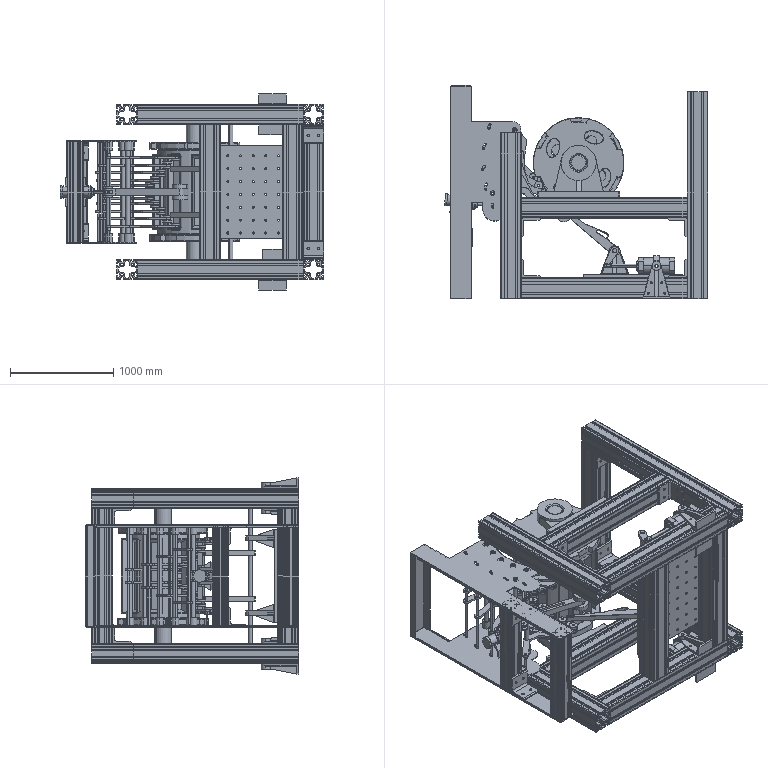Assembly | SolidWorks | mm | 107 component files | 109 solids | 5082 faces | box 2545.98 x 2062 x 1896 mm | volume 839477770 mm3 | plane 3158 | cylinder 1371 | cone 332 | spline 113 | torus 100 | sphere 8 | commonest cylinder face diameters 20 x420 12 x132 24 x88 44.189 x76 60 x61 4 x48 10 x44 85 x40
Bill of materials:
AluminumIngotContainer | 10 |  | Elongated straight prism with a four-sided, non-rectangular (trapezoid/parallelogram-like) cross-section; plain flat faces with no holes or cutouts.
AluminumProfile | 2 |  | Straight extruded bar with a square, slotted profile: two undercut T-style slots on each side, four round bores in the inner lobes, small round corner channels with narrow slits, and a large cross-shaped central cavity.
AluminumProfile100x100 | 6 |  | Straight extruded bar with the same square, slotted profile: two undercut slots per side, four round inner bores, four small corner channels and a cross-shaped central cavity.
AluminumProfile2 | 3 |  | Straight square extruded bar with two undercut slots on each side, four round inner bores, small corner channels and a cross-shaped central cavity; shown standing vertically.
AluminumProfile3 | 2 |  | Straight square extruded bar with two undercut slots on each side, four round inner bores, small corner channels and a cross-shaped central cavity; shown standing vertically.
ConnectingRod1 | 2 | 45 | Flat, thick tapered link plate with rounded ends: a large through-hole in the wide end and a small through-hole in the narrow end.
Cylinder2 | 1 |  | Stepped cylindrical part (shaft or sleeve) with an axial bore. It has end collars, a raised central collar with a radial cross-hole, and a stepped spigot at one end. The bore looks D-shaped, with a flat.
CylinderPistonRod | 2 | 45 | Slender round rod with a flattened eye end (small through-hole) at one end and a larger solid cylindrical head at the other.
cz | 2 |  | Thick circular disc with a small central through-hole and small chamfers on the outer edges and the hole edge.
IngotConnectingArm | 2 | 45 | Flat, elongated, tapered lever plate. It has a rounded boss end with a pivot through-hole, a small radial hole into the boss edge, a triangular through-slot, and a small rectangular tab standing up from one edge.
IngotConnectingRodMandrel | 4 |  | Very long, slender cylindrical rod or tube. The end view shows a central faceted feature that may be a small axial bore or a conical end recess.
IngotSupportRod | 10 | 45 | Thin flat bent link (bell-crank-like) plate with three arm segments, rounded ends, a small hole at each end, and a larger hole at the corner between the first two arms.
Mandrel | 6 | 45 | Long slender cylindrical rod with an enlarged cylindrical collar at each end and a short smaller stub beyond each collar; the end view shows an annular face with a central axial hole.
Mandrel2 | 1 | 45 | Plain solid slender cylindrical rod of uniform diameter with flat ends.
MiddleTrunnionCylinder | 2 | 45 | Axisymmetric body with octagonal prism sections at both ends and a larger octagonal collar in the middle, joined by cylindrical sections, plus a short chamfered cylindrical spigot at one end. A single radial cross-hole passes through the central collar.
MountingPlate | 1 | 45 | Thin flat rectangular plate with a regular grid of small round through holes: 7 rows, where the five inner rows have 9 holes and the top and bottom rows have 7 holes (the two right-hand columns are missing in those rows).
Piston2 | 1 |  | Stepped pin with a larger cylindrical head, a long slender cylindrical shank, and a rounded tip end with a transverse through hole.
Roller | 20 | 45 | Thick circular disc or washer-like ring with a central through hole and chamfered outer edges on both faces.
SmallPin | 2 |  | Stepped cylindrical shaft with a long shank, a larger-diameter collar near one end, and a short smaller stub beyond the collar. The stub end face has a small central hole.
SupportBase | 2 | 45 | Bracket made of a rectangular mounting flange with four small through holes near its ends, and a perpendicular tapered lug with a rounded end and one large through hole.
SupportBase2 | 2 |  | Bracket with a flat rectangular back plate and a perpendicular tapered, pocketed lug. The lug has a raised perimeter rim, a central rib, and a rounded boss at the apex with a through hole.
SupportBase3 | 2 |  | Tapered triangular plate bracket with a rounded apex holding a larger through hole, four smaller through holes in two pairs, and a perpendicular flange along the wide base edge.
SupportBase3 | 1 |  | L-shaped bracket. A flat, symmetric, tapered (trapezoidal) base plate has a wide end and a narrow end with a rounded tip. A rectangular vertical flange rises along the full width of the wide end. A raised central rib runs along the plate's centerline and slopes down from the flange to a thicker cylindrical boss at the narrow end. The boss has a through hole. There are four smaller through holes in the plate, two on each side of the rib.
SupportBase3 | 1 |  | Asymmetric tapered plate bracket. It is a flat plate with one straight side and one angled side, narrowing to a rounded tip. The tip carries a larger through hole in a cylindrical boss that is deeper than the plate. A narrow flange turns down along the wide end. There are four smaller through holes in the plate. The side view suggests a tapered web or gusset under the plate, running from the flange to the boss.
SupportBase4 | 2 |  | Triangular gusset-style bracket: a triangular plate with a rounded apex and one through hole, joined at its base to a perpendicular rectangular flange that has two through holes.
SupportFrame | 1 |  | Thin-walled C-shaped frame: two parallel long thin strips joined at one end by a perpendicular web. Each strip has a lobed side extension with a concave curved edge, a row of round holes, and a row of short arc-shaped slots.
TappingArm | 1 |  | Long, flat, straight lever arm. One end has a cylindrical hub with a through bore, and a forked side lug extends from that end at an angle. The arm has a long slot along its length and a small hole near its rounded far end.
U-shapedPlate | 12 |  | L-section angle bracket with two legs of similar length at 90 degrees. It has a rounded inner bend, slightly rounded outer corner and chamfered leg tips. Each leg has two round through-holes in a line.
Wheel | 1 | 45 | Short solid cylinder with a central axial bore and four smaller axial through-holes evenly spaced on a bolt circle. The outer surface has longitudinal rectangular recessed pockets around its circumference, and the end edges are chamfered.
WheelIndexingPlate | 2 | 45 | Thin flat disc with a stepped, notched outer edge, a central round hole, and four oval through-holes arranged around the center.
WheelMandrel | 1 |  | Plain solid straight cylindrical rod or pin with small chamfers at both ends.
Mates:
1. coincident | SupportFrame-2 plane at (0, 0, 0) dir (0, 0, 1) | assembly plane at (0, 0, 0) dir (0, 0, 1)
2. coincident | SupportFrame-2 plane at (0, 0, 0) dir (0, 1, 0) | assembly plane at (0, 0, 0) dir (0, 1, 0)
3. coincident | SupportFrame-2 plane at (0, 0, 0) dir (1, 0, 0) | assembly plane at (0, 0, 0) dir (1, 0, 0)
4. width | Wheel-1 face at (1138.564, 280.356, 80) dir (0, 0, -1) | Wheel-1 face at (1138.564, 280.356, 910) dir (0, 0, 1) | SupportFrame-2 face at (0, 0, 0) dir (0, 0, -1) | SupportFrame-2 face at (0, 0, 990) dir (0, 0, 1)
5. concentric | SupportFrame-2 face at (521.144, 598.058, -1429) dir (0, 0, 1) r 22.094 | Mandrel-1 face at (521.144, 598.058, 995) dir (0, 0, -1) r 22.094
6. width | Mandrel-1 face at (521.144, 598.058, -5) dir (0, 0, -1) | Mandrel-1 face at (521.144, 598.058, 995) dir (0, 0, 1) | SupportFrame-2 face at (0, 0, 990) dir (0, 0, 1) | SupportFrame-2 face at (0, 0, 0) dir (0, 0, -1)
7. concentric | Wheel-1 face at (1138.564, 280.356, -180) dir (0, 0, 1) r 80 | SupportBase-1 face at (1138.564, 280.356, -155) dir (0, 0, -1) r 80
8. concentric | Mandrel-1 face at (521.144, 598.058, 995) dir (0, 0, -1) r 22.094 | IngotSupportRod-1 face at (521.144, 598.058, 445) dir (0, 0, -1) r 22.094
9. concentric | IngotSupportRod-1 face at (705.127, 143.342, 445) dir (0, 0, -1) r 30 | Roller-2 face at (705.127, 143.342, 470) dir (0, 0, -1) r 10
10. concentric | IngotSupportRod-1 face at (705.127, 143.342, 445) dir (0, 0, -1) r 30 | Roller-1 face at (705.127, 143.342, 425) dir (0, 0, -1) r 10
11. coincident | IngotSupportRod-1 face at (17.945, 67.185, 425) dir (0, 0, -1) | Roller-1 face at (705.127, 143.342, 425) dir (0, 0, 1)
12. coincident | IngotSupportRod-1 face at (17.945, 67.185, 445) dir (0, 0, 1) | Roller-2 face at (705.127, 143.342, 445) dir (0, 0, -1)
13. concentric | Mandrel-4 face at (440.739, 312.216, 995) dir (0, 0, -1) r 22.094 | IngotSupportRod-5 face at (440.739, 312.216, 320) dir (0, 0, -1) r 22.094
14. concentric | Mandrel-5 face at (450.613, 163.114, 995) dir (0, 0, -1) r 22.094 | IngotSupportRod-6 face at (450.613, 163.114, 245) dir (0, 0, -1) r 22.094
15. concentric | Mandrel-6 face at (493.776, 20.056, 995) dir (0, 0, -1) r 22.094 | IngotSupportRod-7 face at (493.776, 20.056, 170) dir (0, 0, -1) r 22.094
16. concentric | Roller-3 face at (753.229, 63.053, 370) dir (0, 0, -1) r 10 | IngotSupportRod-4 face at (753.229, 63.053, 390) dir (0, 0, -1) r 10
17. coincident | Roller-3 face at (753.229, 63.053, 370) dir (0, 0, 1) | IngotSupportRod-4 face at (104.912, -177.165, 370) dir (0, 0, -1)
18. concentric | Roller-3 face at (753.229, 63.053, 370) dir (0, 0, -1) r 42.5 | Roller-7 face at (753.229, 63.053, 415) dir (0, 0, -1) r 42.5
19. coincident | Roller-7 face at (753.229, 63.053, 390) dir (0, 0, -1) | IngotSupportRod-4 face at (104.912, -177.165, 390) dir (0, 0, 1)
20. concentric | Roller-4 face at (809.993, -10.688, 345) dir (0, 0, -1) r 42.5 | Roller-8 face at (809.993, -10.688, 300) dir (0, 0, -1) r 42.5
21. concentric | Roller-4 face at (809.993, -10.688, 345) dir (0, 0, -1) r 42.5 | IngotSupportRod-5 face at (809.993, -10.688, 320) dir (0, 0, -1) r 30
22. coincident | Roller-4 face at (809.993, -10.688, 320) dir (0, 0, -1) | IngotSupportRod-5 face at (230.978, -388.524, 320) dir (0, 0, 1)
23. coincident | Roller-8 face at (809.993, -10.688, 300) dir (0, 0, 1) | IngotSupportRod-5 face at (230.978, -388.524, 300) dir (0, 0, -1)
24. concentric | Roller-5 face at (870.434, -90.592, 270) dir (0, 0, -1) r 10 | IngotSupportRod-6 face at (870.434, -90.592, 245) dir (0, 0, -1) r 30
25. coincident | Roller-5 face at (870.434, -90.592, 245) dir (0, 0, -1) | IngotSupportRod-6 face at (366.019, -563.439, 245) dir (0, 0, 1)
26. concentric | Roller-9 face at (870.434, -90.592, 225) dir (0, 0, -1) r 10 | IngotSupportRod-6 face at (870.434, -90.592, 245) dir (0, 0, -1) r 30
27. coincident | Roller-9 face at (870.434, -90.592, 225) dir (0, 0, 1) | IngotSupportRod-6 face at (366.019, -563.439, 225) dir (0, 0, -1)
28. concentric | Roller-6 face at (950.087, -159.933, 195) dir (0, 0, -1) r 42.5 | Roller-10 face at (950.087, -159.933, 150) dir (0, 0, -1) r 42.5
29. concentric | Roller-6 face at (950.087, -159.933, 195) dir (0, 0, -1) r 42.5 | IngotSupportRod-7 face at (950.087, -159.933, 170) dir (0, 0, -1) r 30
30. coincident | Roller-6 face at (950.087, -159.933, 170) dir (0, 0, -1) | IngotSupportRod-7 face at (531.776, -710.418, 170) dir (0, 0, 1)
31. coincident | Roller-10 face at (950.087, -159.933, 150) dir (0, 0, 1) | IngotSupportRod-7 face at (531.776, -710.418, 150) dir (0, 0, -1)
32. concentric | Wheel-1 face at (1138.564, 280.356, -180) dir (0, 0, 1) r 80 | WheelIndexingPlate-1 face at (1138.564, 280.356, 80) dir (0, 0, -1) r 80
33. coincident | Wheel-1 face at (1138.564, 280.356, 80) dir (0, 0, -1) | WheelIndexingPlate-1 face at (1138.564, 280.356, 80) dir (0, 0, 1)
34. concentric | Mandrel-3 face at (464.658, 459.717, 995) dir (0, 0, -1) r 22.094 | IngotSupportRod-4 face at (464.658, 459.717, 390) dir (0, 0, -1) r 22.094
35. concentric | Wheel-1 face at (1138.564, 280.356, 910) dir (0, 0, -1) r 357.5 | WheelIndexingPlate-3 face at (1138.564, 280.356, 970) dir (0, 0, -1) r 395
36. coincident | Wheel-1 face at (1138.564, 280.356, 910) dir (0, 0, 1) | WheelIndexingPlate-3 face at (1138.564, 280.356, 910) dir (0, 0, -1)
37. coincident | Wheel-1 face at (925.229, 626.929, 135) dir (-0.9256, -0.3784, 0) | AluminumIngotContainer-1 face at (925.229, 626.929, 135) dir (0.9256, 0.3784, 0)
38. coincident | Wheel-1 face at (919.439, 521.727, 80) dir (-0.6722, 0.7404, 0) | AluminumIngotContainer-1 face at (919.439, 521.727, 495) dir (0.6722, -0.7404, 0)
39. coincident | Wheel-1 face at (925.229, 626.929, 855) dir (-0.2299, 0.2532, -0.9397) | AluminumIngotContainer-1 face at (814.168, 526.105, 855) dir (0.2299, -0.2532, 0.9397)
40. concentric | MiddleTrunnionCylinder-1 face at (1766, -713.926, -260) dir (-1, 0.0005394, 0) r 40 | CylinderPistonRod-1 face at (1749.707, -713.917, -260) dir (1, -0.0005394, 0) r 40
41. parallel | MiddleTrunnionCylinder-1 face at (1765.96, -788.926, -335) dir (0, 0, -1) | CylinderPistonRod-1 face at (1399.707, -713.728, -280) dir (0, 0, -1)
42. concentric | CylinderPistonRod-1 face at (1399.707, -713.728, -280) dir (0, 0, 1) r 8.5 | ConnectingRod1-1 face at (1399.707, -713.728, -200) dir (0, 0, -1) r 8.5
43. distance | IngotSupportRod-1 face at (17.945, 67.185, 445) dir (0, 0, 1) | IngotSupportRod-13 face at (17.945, 67.185, 545) dir (0, 0, -1)
44. distance | IngotSupportRod-4 face at (104.912, -177.165, 390) dir (0, 0, 1) | IngotSupportRod-12 face at (104.912, -177.165, 600) dir (0, 0, -1)
45. distance | IngotSupportRod-5 face at (230.978, -388.524, 320) dir (0, 0, 1) | IngotSupportRod-16 face at (230.978, -388.524, 670) dir (0, 0, -1)
46. distance | IngotSupportRod-6 face at (366.019, -563.439, 245) dir (0, 0, 1) | IngotSupportRod-15 edge at (458.04, 192.181, 745) dir (0.9689, -0.2475, 0)
47. distance | IngotSupportRod-7 face at (531.776, -710.418, 170) dir (0, 0, 1) | IngotSupportRod-14 face at (531.776, -710.418, 820) dir (0, 0, -1)
48. coincident | CylinderPistonRod-1 face at (1399.707, -713.728, -240) dir (0, 0, 1) | ConnectingRod1-1 face at (468.852, 496.589, -240) dir (0, 0, -1)
49. concentric | ConnectingRod1-1 face at (1486.2, -567.376, -200) dir (0, 0, -1) r 21.5 | Mandrel2-1 face at (1486.2, -567.376, 748.53) dir (0, 0, -1) r 21.5
50. concentric | Mandrel2-1 face at (1486.2, -567.376, 748.53) dir (0, 0, -1) r 21.5 | IngotConnectingArm-1 face at (1486.2, -567.376, 297.813) dir (0, 0, -1) r 21.5
51. coincident | AluminumProfile100x100-1 face at (2186, -968.8, -155) dir (0, 0, 1) | AluminumProfile100x100-3 face at (2186, -190.8, -155) dir (0, 0, 1)
52. coincident | AluminumProfile100x100-2 face at (448.2, 569, -355) dir (0, 0, -1) | AluminumProfile100x100-3 face at (2186, -115.2, -355) dir (0, 0, -1)
53. coincident | AluminumProfile100x100-2 face at (586, 569, -292.8) dir (1, 0, 0) | AluminumProfile100x100-3 face at (586, -248, -350) dir (-1, 0, 0)
54. coincident | AluminumProfile100x100-1 face at (586, -1026, -160) dir (-1, 0, 0) | AluminumProfile100x100-2 face at (586, 569, -292.8) dir (1, 0, 0)
55. coincident | SupportFrame-2 face at (100, -1031, 10) dir (0, -1, 0) | AluminumProfile100x100-2 face at (391, -1031, -350) dir (0, -1, 0)
56. parallel | SupportFrame-2 face at (100, -1031, 10) dir (0, -1, 0) | SupportBase-1 face at (138.564, -53, -155) dir (0, -1, 0)
57. coincident | SupportBase-1 face at (138.564, -53, -155) dir (0, -1, 0) | AluminumProfile100x100-3 face at (2186, -53, -217.2) dir (0, 1, 0)
58. coincident | SupportBase-1 face at (138.564, 0.2627, -155) dir (0, 0, 1) | AluminumProfile100x100-3 face at (2186, -90.8, -155) dir (0, 0, 1)
59. distance | Wheel-1 plane at (1138.564, 280.356, 495) dir (0, 0, 1) | AluminumProfile100x100-3 face at (2186, -190.8, -155) dir (0, 0, 1)
60. coincident | AluminumProfile100x100-1 face at (2186, -1026, -160) dir (1, 0, 0) | AluminumProfile-1 face at (2186, 969, -217.2) dir (-1, 0, 0)
61. coincident | AluminumProfile100x100-1 face at (2186, -1031, -292.8) dir (0, -1, 0) | AluminumProfile-1 face at (2191, -1031, -350) dir (0, -1, 0)
62. coincident | AluminumProfile100x100-1 face at (2186, -1031, -292.8) dir (0, -1, 0) | AluminumProfile2-1 face at (2123.8, -1031, 1145) dir (0, -1, 0)
63. coincident | AluminumProfile100x100-5 face at (2186, -1031, 1207.2) dir (0, -1, 0) | AluminumProfile100x100-6 face at (391, -1031, 1150) dir (0, -1, 0)
64. coincident | AluminumProfile100x100-5 face at (2186, -893.2, 1145) dir (0, 0, -1) | AluminumProfile2-1 face at (1991, -1026, 1145) dir (0, 0, 1)
65. coincident | MiddleTrunnionCylinder-1 face at (1915.976, -759.007, -355) dir (0, 0, -1) | AluminumProfile100x100-1 face at (2186, -893.2, -355) dir (0, 0, -1)
66. coincident | MountingPlate-1 face at (-545.911, -831, -80.281) dir (0, -1, 0) | AluminumProfile2-1 face at (2048.2, -831, 1145) dir (0, 1, 0)
67. coincident | MountingPlate-1 face at (2186, -801, 45) dir (1, 0, 0) | AluminumProfile2-1 face at (2186, -893.2, 1145) dir (1, 0, 0)
68. distance | SupportBase-1 face at (742.414, 0.2627, -155) dir (-1, 0, 0) | AluminumProfile100x100-2 face at (586, 569, -292.8) dir (1, 0, 0)
69. coincident | AluminumProfile100x100-3 face at (2186, -115.2, -355) dir (0, 0, -1) | AluminumProfile-1 face at (2248.2, 969, -355) dir (0, 0, -1)
70. distance | SupportBase-1 face at (138.564, -53, -155) dir (0, -1, 0) | AluminumProfile100x100-1 face at (2186, -1031, -292.8) dir (0, -1, 0)
71. coincident | AluminumProfile100x100-1 face at (2186, -968.8, -155) dir (0, 0, 1) | AluminumProfile2-2 face at (1191, -836, -155) dir (0, 0, -1)
72. coincident | AluminumProfile100x100-1 face at (2186, -1031, -292.8) dir (0, -1, 0) | AluminumProfile2-2 face at (1323.8, -1031, 1145) dir (0, -1, 0)
73. coincident | MountingPlate-1 face at (1186, -801, 45) dir (-1, 0, 0) | AluminumProfile2-2 face at (1186, -968.8, 1145) dir (-1, 0, 0)
74. coincident | AluminumProfile-1 face at (2186, 969, -217.2) dir (-1, 0, 0) | AluminumProfile2-1 face at (2186, -893.2, 1145) dir (1, 0, 0)
75. coincident | MountingPlate-1 face at (-545.911, -801, -80.281) dir (0, 1, 0) | SupportBase2-2 face at (165.227, -801, 120) dir (0, -1, 0)
76. concentric | Mandrel2-1 face at (1486.2, -567.376, 748.53) dir (0, 0, -1) r 21.5 | SupportBase2-2 face at (1486.2, -567.376, 120) dir (0, 0, 1) r 21.5
77. coincident | MountingPlate-1 face at (2186, -801, 45) dir (0, 0, -1) | SupportBase2-2 face at (165.227, 0, 45) dir (0, 0, -1)
78. distance | AluminumProfile100x100-2 face at (386, 569, -217.2) dir (-1, 0, 0) | SupportFrame-2 face at (-100, 1031, 10) dir (-1, 0, 0)
79. width | AluminumProfile100x100-1 face at (2186, -893.2, -355) dir (0, 0, -1) | AluminumProfile100x100-5 face at (2186, -968.8, 1345) dir (0, 0, 1) | MountingPlate-1 face at (2186, -801, 45) dir (0, 0, -1) | MountingPlate-1 face at (2186, -801, 945) dir (0, 0, 1)
80. distance | AluminumProfile2-2 face at (1346.2, -841, 1145) dir (-1, 0, 0) | SupportBase2-2 face at (1466.2, -659.188, 133) dir (-1, 0, 0)
81. coincident | AluminumProfile100x100-1 face at (2186, -1031, -292.8) dir (0, -1, 0) | SupportBase3-1 face at (1336.2, -1031, -375) dir (0, -1, 0)
82. concentric | MiddleTrunnionCylinder-1 face at (1891, -713.993, -415) dir (0, 0, 1) r 15 | SupportBase3-1 face at (1891, -713.993, -375) dir (0, 0, 1) r 15
83. distance | SupportBase3-1 face at (1906, -850.78, -404) dir (1, 0, 0) | AluminumProfile-1 face at (2386, 969, -292.8) dir (1, 0, 0)
84. parallel | ConnectingRod1-1 face at (1675.336, -366.804, -200) dir (0.8132, -0.582, 0) | IngotConnectingArm-1 face at (1107.928, -241.338, 297.813) dir (0.8132, -0.582, 0)
85. concentric | MiddleTrunnionCylinder-1 face at (1891, -713.993, -415) dir (0, 0, 1) r 15 | SupportBase3-2 face at (1891, -713.993, -135) dir (0, 0, -1) r 15
86. coincident | AluminumProfile100x100-1 face at (2186, -1031, -292.8) dir (0, -1, 0) | SupportBase3-2 face at (2445.8, -1031, -135) dir (0, -1, 0)
87. coincident | AluminumProfile100x100-1 face at (2186, -1026, -155) dir (0, 0, 1) | SupportBase3-2 face at (2445.8, -908.993, -155) dir (0, 0, -1)
88. concentric | Mandrel2-1 face at (1492.399, -572.235, 272.813) dir (-0.7871, 0.6169, 0) r 8 | IngotConnectingArm-1 face at (1521.618, -595.136, 272.813) dir (0.7871, -0.6169, 0) r 8
89. width | AluminumProfile100x100-5 face at (2186, -968.8, 1345) dir (0, 0, 1) | AluminumProfile100x100-1 face at (2186, -893.2, -355) dir (0, 0, -1) | Mandrel2-1 face at (1486.2, -567.376, -248.47) dir (0, 0, -1) | Mandrel2-1 face at (1486.2, -567.376, 1238.47) dir (0, 0, 1)
90. distance | CylinderPistonRod-1 face at (1799.707, -713.944, -260) dir (1, -0.0005394, 0) | MiddleTrunnionCylinder-1 face at (2016.387, 2.939, -1754.26) dir (-1, 0.0005394, 0)
91. coincident | AluminumProfile100x100-1 face at (2186, -893.2, -355) dir (0, 0, -1) | SupportBase3-1 face at (1336.2, -908.993, -355) dir (0, 0, 1)
92. coincident | SupportFrame-2 face at (0, 0, 980) dir (0, 0, -1) | AluminumProfile3-1 face at (-86.25, -203.572, 980) dir (0, 0, 1)
93. coincident | SupportFrame-2 face at (-90, 926.986, 20) dir (1, 0, 0) | AluminumProfile3-1 face at (-90, -303.172, 980) dir (-1, 0, 0)
94. distance | SupportFrame-2 face at (90, -119.822, 20) dir (0, 1, 0) | AluminumProfile3-1 face at (31.65, -199.822, 980) dir (0, 1, 0)
95. coincident | SupportFrame-2 face at (0, 0, 10) dir (0, 0, 1) | AluminumProfile3-2 face at (-86.25, -884.75, 10) dir (0, 0, -1)
96. coincident | SupportFrame-2 face at (-90, 926.986, 20) dir (1, 0, 0) | AluminumProfile3-2 face at (-90, -984.35, 980) dir (-1, 0, 0)
97. coincident | SupportFrame-2 face at (100, -1031, 10) dir (0, -1, 0) | AluminumProfile3-2 face at (13.35, -1031, 980) dir (0, -1, 0)
98. coincident | AluminumProfile3-1 face at (-43.35, -199.822, 980) dir (0, 1, 0) | SupportBase4-1 face at (19.647, -199.822, 632.958) dir (0, -1, 0)
99. concentric | Cylinder2-1 face at (-15, -91.375, 405) dir (0, 0, 1) r 11.5 | SupportBase4-1 face at (-15, -91.375, 437.28) dir (0, 0, -1) r 11.5
100. width | AluminumProfile3-1 face at (-90, -303.172, 980) dir (-1, 0, 0) | AluminumProfile3-1 face at (60, -246.472, 980) dir (1, 0, 0) | SupportBase4-1 face at (-25, -130.511, 397.53) dir (-1, 0, 0) | SupportBase4-1 face at (-5, -130.511, 397.53) dir (1, 0, 0)
101. concentric | Cylinder2-1 face at (144.994, -111.29, 495) dir (-0.9923, 0.1235, 0) r 50 | Piston2-1 face at (257.687, -125.317, 495) dir (-0.9923, 0.1235, 0) r 15
102. concentric | SupportFrame-2 face at (306.906, -12.931, 990) dir (0, 0, -1) r 22.095 | Mandrel-7 face at (306.906, -12.931, 995) dir (0, 0, -1) r 22.094
103. coincident | SupportFrame-2 face at (0, 0, 980) dir (0, 0, -1) | Mandrel-7 face at (306.906, -12.931, 980) dir (0, 0, 1)
104. concentric | TappingArm-1 face at (306.906, -12.931, 525) dir (0, 0, -1) r 22.095 | Mandrel-7 face at (306.906, -12.931, 995) dir (0, 0, -1) r 22.094
105. concentric | Piston2-1 face at (302.342, -130.875, 510) dir (0, 0, -1) r 8 | TappingArm-1 face at (302.342, -130.875, 525) dir (0, 0, -1) r 8
106. coincident | Piston2-1 face at (302.342, -130.875, 510) dir (0, 0, 1) | TappingArm-1 face at (4.467, 40.819, 510) dir (0, 0, -1)
107. width | SupportFrame-2 face at (0, 0, 990) dir (0, 0, 1) | SupportFrame-2 face at (0, 0, 0) dir (0, 0, -1) | SupportBase4-1 face at (19.647, -70.838, 412.28) dir (0, 0, -1) | SupportBase4-2 face at (-49.647, -70.838, 577.72) dir (0, 0, 1)
108. concentric | TappingArm-1 face at (997.956, -215.048, 525) dir (0, 0, -1) r 36 | cz-1 face at (997.956, -215.048, 465) dir (0, 0, -1) r 75
109. coincident | TappingArm-1 face at (4.467, 40.819, 465) dir (0, 0, -1) | cz-1 face at (997.956, -215.048, 465) dir (0, 0, 1)
110. concentric | TappingArm-1 face at (997.956, -215.048, 525) dir (0, 0, -1) r 36 | cz-2 face at (997.956, -215.048, 571) dir (0, 0, -1) r 75
111. coincident | TappingArm-1 face at (4.467, 40.819, 525) dir (0, 0, 1) | cz-2 face at (997.956, -215.048, 525) dir (0, 0, -1)
112. coincident | AluminumProfile-1 face at (2191, 969, -350) dir (0, 1, 0) | AluminumProfile2-4 face at (2248.2, 969, 1145) dir (0, 1, 0)
113. coincident | AluminumProfile-1 face at (2386, 969, -292.8) dir (1, 0, 0) | AluminumProfile2-4 face at (2386, 906.8, 1145) dir (1, 0, 0)
114. coincident | AluminumProfile-1 face at (2323.8, 969, -155) dir (0, 0, 1) | AluminumProfile2-4 face at (2191, 774, -155) dir (0, 0, -1)
115. concentric | SupportBase-2 face at (1138.564, 280.356, 1145) dir (0, 0, 1) r 80 | WheelMandrel-1 face at (1138.564, 280.356, -255) dir (0, 0, 1) r 80
116. width | SupportBase-1 face at (1138.564, 280.356, -265) dir (0, 0, -1) | SupportBase-2 face at (1138.564, 280.356, 1255) dir (0, 0, 1) | WheelMandrel-1 face at (1138.564, 280.356, -255) dir (0, 0, -1) | WheelMandrel-1 face at (1138.564, 280.356, 1245) dir (0, 0, 1)
117. slot | IngotConnectingRodMandrel-1 face at (271.039, 615.177, -1.5) dir (0, 0, 1) r 10 | SupportFrame-2 face at (335.837, 614.405, 1660) dir (0, 0, -1) r 53.682
118. concentric | IngotSupportRod-1 face at (271.039, 615.177, 425) dir (0, 0, 1) r 10 | IngotConnectingRodMandrel-1 face at (271.039, 615.177, -1.5) dir (0, 0, 1) r 10
119. width | IngotConnectingRodMandrel-1 face at (271.039, 615.177, -1.5) dir (0, 0, -1) | IngotConnectingRodMandrel-1 face at (271.039, 615.177, 991.5) dir (0, 0, 1) | SupportFrame-2 face at (0, 0, 990) dir (0, 0, 1) | SupportFrame-2 face at (0, 0, 0) dir (0, 0, -1)
120. concentric | SupportFrame-2 face at (217.846, 415.792, 1660) dir (0, 0, -1) r 10.524 | IngotConnectingRodMandrel-2 face at (217.846, 415.792, 0) dir (0, 0, 1) r 10
121. coincident | SupportFrame-2 face at (0, 0, 0) dir (0, 0, -1) | IngotConnectingRodMandrel-2 face at (217.846, 415.792, 0) dir (0, 0, -1)
122. concentric | SupportFrame-2 face at (209.784, 214.72, 1660) dir (0, 0, -1) r 10.015 | IngotConnectingRodMandrel-3 face at (209.784, 214.72, 0) dir (0, 0, 1) r 10
123. coincident | SupportFrame-2 face at (0, 0, 0) dir (0, 0, -1) | IngotConnectingRodMandrel-3 face at (209.784, 214.72, 0) dir (0, 0, -1)
124. coincident | SupportFrame-2 face at (0, 0, 0) dir (0, 0, -1) | IngotConnectingRodMandrel-4 face at (240.154, 26.908, 0) dir (0, 0, -1)
125. concentric | SupportFrame-2 face at (240.154, 26.908, 1660) dir (0, 0, -1) r 10.764 | IngotConnectingRodMandrel-4 face at (240.154, 26.908, 993) dir (0, 0, -1) r 10
126. coincident | AluminumProfile-1 face at (2186, 969, -217.2) dir (-1, 0, 0) | U-shapedPlate-1 face at (2186, -433, -155) dir (1, 0, 0)
127. coincident | AluminumProfile-1 face at (2191, 969, -355) dir (0, 0, -1) | U-shapedPlate-1 face at (2146, -293, -355) dir (0, 0, -1)
128. coincident | AluminumProfile100x100-3 face at (2186, -253, -292.8) dir (0, -1, 0) | U-shapedPlate-1 face at (2186, -253, -155) dir (0, 1, 0)
129. coincident | AluminumProfile2-4 face at (2386, 906.8, 1145) dir (1, 0, 0) | U-shapedPlate-3 face at (2386, 729, -115) dir (1, 0, 0)
130. coincident | AluminumProfile2-4 face at (2323.8, 769, 1145) dir (0, -1, 0) | U-shapedPlate-3 face at (2386, 769, -155) dir (0, 1, 0)
131. coincident | AluminumProfile-1 face at (2323.8, 969, -155) dir (0, 0, 1) | U-shapedPlate-3 face at (2386, 589, -155) dir (0, 0, -1)
132. coincident | AluminumProfile100x100-2 face at (586, 569, -292.8) dir (1, 0, 0) | U-shapedPlate-4 face at (586, -433, -355) dir (-1, 0, 0)
133. coincident | AluminumProfile100x100-3 face at (2186, -253, -292.8) dir (0, -1, 0) | U-shapedPlate-4 face at (586, -253, -355) dir (0, 1, 0)
134. coincident | AluminumProfile100x100-2 face at (448.2, 569, -355) dir (0, 0, -1) | U-shapedPlate-4 face at (626, -293, -355) dir (0, 0, -1)
135. coincident | AluminumProfile100x100-2 face at (586, 569, -292.8) dir (1, 0, 0) | U-shapedPlate-5 face at (586, -831, -355) dir (-1, 0, 0)
136. coincident | AluminumProfile100x100-2 face at (448.2, 569, -355) dir (0, 0, -1) | U-shapedPlate-5 face at (626, -791, -355) dir (0, 0, -1)
137. coincident | AluminumProfile100x100-1 face at (2186, -831, -217.2) dir (0, 1, 0) | U-shapedPlate-5 face at (766, -831, -355) dir (0, -1, 0)
138. coincident | AluminumProfile-1 face at (2186, 969, -217.2) dir (-1, 0, 0) | U-shapedPlate-6 face at (2186, -831, -155) dir (1, 0, 0)
139. coincident | AluminumProfile-1 face at (2248.2, 969, -355) dir (0, 0, -1) | U-shapedPlate-6 face at (2146, -791, -355) dir (0, 0, -1)
140. coincident | AluminumProfile100x100-1 face at (2186, -831, -217.2) dir (0, 1, 0) | U-shapedPlate-6 face at (2006, -831, -155) dir (0, -1, 0)
141. coincident | AluminumProfile3-1 face at (13.35, -349.822, 980) dir (0, -1, 0) | U-shapedPlate-12 face at (110, -349.822, 10) dir (0, 1, 0)
142. coincident | AluminumProfile3-1 face at (-90, -303.172, 980) dir (-1, 0, 0) | U-shapedPlate-12 face at (-90, -389.822, 50) dir (-1, 0, 0)
143. coincident | SupportFrame-2 face at (0, 0, 10) dir (0, 0, 1) | U-shapedPlate-12 face at (110, -529.822, 10) dir (0, 0, -1)
144. concentric | IngotSupportRod-7 face at (309.034, -149.403, 150) dir (0, 0, 1) r 10 | SmallPin-2 face at (309.034, -149.403, 170) dir (0, 0, -1) r 10
145. coincident | SupportFrame-2 face at (0, 0, 0) dir (0, 0, -1) | SmallPin-2 face at (309.034, -149.403, 0) dir (0, 0, -1)
146. distance | SupportBase4-1 face at (19.647, -70.838, 437.28) dir (0, 0, 1) | Cylinder2-1 face at (-65.293, -19.613, 437.5) dir (0, 0, -1)